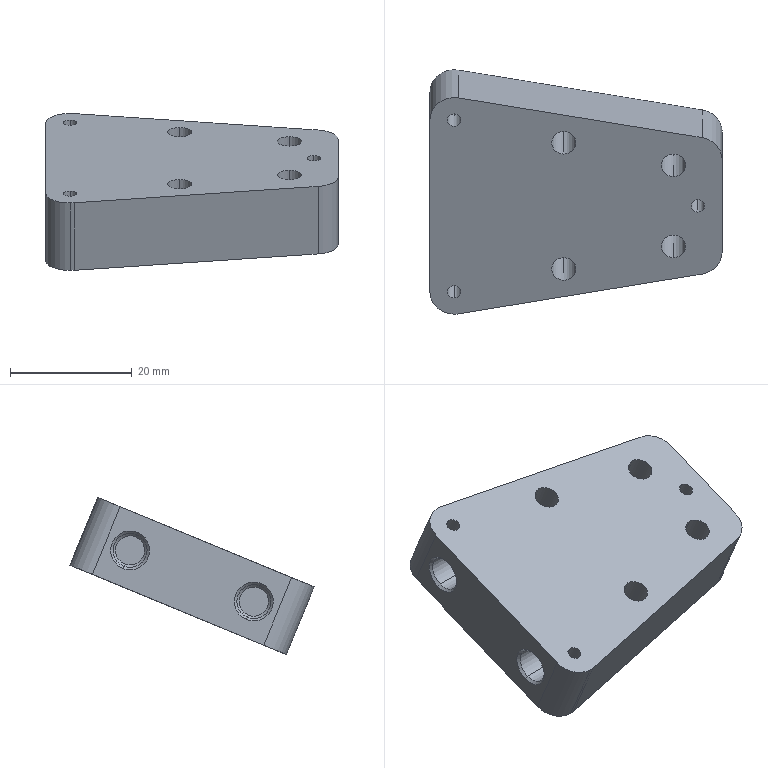Component | SolidWorks | Holding Part-1 | 1 solid | 39 faces | box 48 x 40.13 x 25.78 mm | volume 16952 mm3 | cylinder 23 | cone 8 | plane 8 | commonest cylinder face diameters 4 x8 2.2 x6 8 x5 5.6 x4
build123d program:
from build123d import *

# Parameters (mm, degrees)
SKETCH2_R           = 2.75
SKETCH2_R_2         = 5
BOSS_EXTRUDE1_DEPTH = 15
SKETCH1_R           = 7
CUT_EXTRUDE1_DEPTH  = 15
CHAMFER1_SIZE       = 1
SCALE1_SCALE        = 0.4


with BuildPart() as part:
    # Sketch2 → Boss-Extrude1 (new, symmetric)
    with BuildSketch(Plane.XY):
        with BuildLine():
            Line((-38.082, 120), (38.082, 120))
            ThreePointArc((38.082, 120), (45.742, 116.428), (47.93, 108.264))
            Line((47.93, 108.264), (30.297, 8.264))
            ThreePointArc((30.297, 8.264), (26.877, 2.34), (20.449, 0))
            Line((20.449, 0), (-20.449, 0))
            ThreePointArc((-20.449, 0), (-26.877, 2.34), (-30.297, 8.264))
            Line((-30.297, 8.264), (-47.93, 108.264))
            ThreePointArc((-47.93, 108.264), (-45.742, 116.428), (-38.082, 120))
        make_face()
        with Locations((38.082, 110)):
            Circle(SKETCH2_R, mode=Mode.SUBTRACT)
        with Locations((18, 20)):
            Circle(SKETCH2_R_2, mode=Mode.SUBTRACT)
        with Locations((28, 65)):
            Circle(SKETCH2_R_2, mode=Mode.SUBTRACT)
        with Locations((0, 10)):
            Circle(SKETCH2_R, mode=Mode.SUBTRACT)
        with Locations(Location((-18, 20, 0), (0, 0, 180))):
            Circle(SKETCH2_R_2, mode=Mode.SUBTRACT)
        with Locations(Location((-28, 65, 0), (0, 0, 180))):
            Circle(SKETCH2_R_2, mode=Mode.SUBTRACT)
        with Locations(Location((-38.082, 110, 0), (0, 0, 180))):
            Circle(SKETCH2_R, mode=Mode.SUBTRACT)
    extrude(amount=BOSS_EXTRUDE1_DEPTH, both=True)

    # Sketch1 → Cut-Extrude1 (cut)
    with BuildSketch(Plane(origin=(0, 120, 0), x_dir=(1, 0, 0), z_dir=(0, 1, 0))):
        with Locations(Location((-27.5, 0, 0), (0, 0, 270))):
            Circle(SKETCH1_R)
        with Locations(Location((27.5, 0, 0), (0, 0, 90))):
            Circle(SKETCH1_R)
    extrude(amount=-CUT_EXTRUDE1_DEPTH, mode=Mode.SUBTRACT)

    # Chamfer1
    chamfer1_edges = [part.edges().sort_by_distance(p)[0] for p in [
        (-27.5, 105, -7),
        (-27.5, 120, -7),
        (27.5, 105, 7),
        (27.5, 120, 7),
    ]]
    chamfer(chamfer1_edges, length=CHAMFER1_SIZE)


with BuildPart() as part_1:
    # Scale1: scaled about (0, 0, 0)
    add(part.part.scale(SCALE1_SCALE))


solid = part_1.part

# Placed as in the assembly
solid = solid.moved(Location((346.621, -9.012, 55.479), (-157.552, 0, 90)))